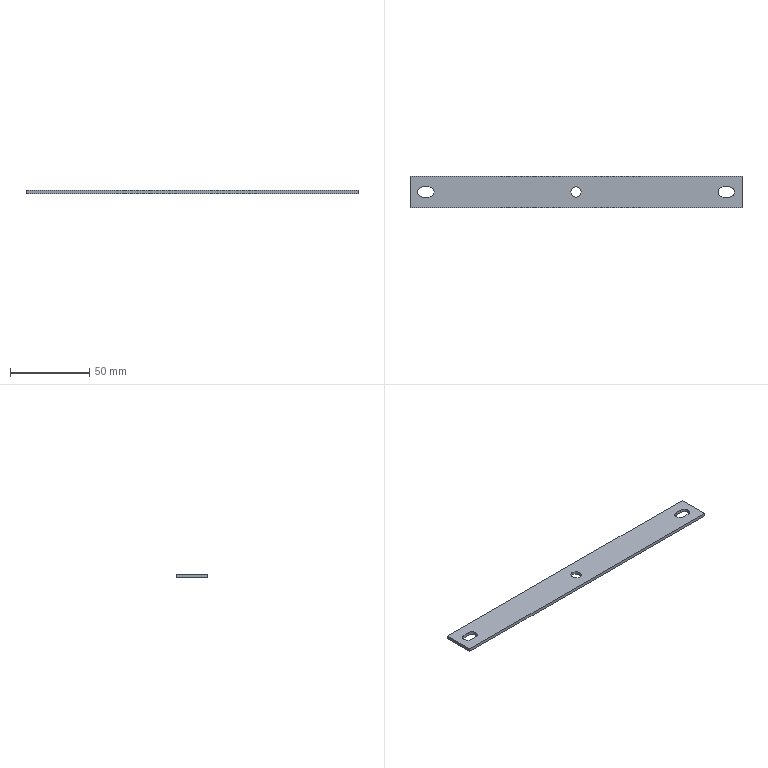Component | SolidWorks | FanFixingPlate-1 | 1 solid | 18 faces | box 210 x 20 x 2 mm | volume 8103 mm3 | plane 10 | cylinder 8 | commonest cylinder face diameters 6.4 x6 6.5 x2
build123d program:
from build123d import *

# Parameters (mm, degrees)
SKETCH1_W           = 210
SKETCH1_H           = 20
BOSS_EXTRUDE1_DEPTH = 1
SKETCH2_R           = 3.25
CUT_EXTRUDE1_DEPTH  = 2


with BuildPart() as part:
    # Sketch1 → Boss-Extrude1 (new, symmetric)
    with BuildSketch(Plane.XY):
        Rectangle(SKETCH1_W, SKETCH1_H)
    extrude(amount=BOSS_EXTRUDE1_DEPTH, both=True)

    # Sketch2 → Cut-Extrude1 (cut)
    with BuildSketch(Plane.XY.offset(1)):
        Circle(SKETCH2_R)
        with BuildLine():
            Line((-97, 3.2), (-93, 3.2))
            ThreePointArc((-93, 3.2), (-89.8, 0), (-93, -3.2))
            Line((-93, -3.2), (-97, -3.2))
            ThreePointArc((-97, -3.2), (-100.2, 0), (-97, 3.2))
        make_face()
        with BuildLine():
            Line((97, 3.2), (93, 3.2))
            ThreePointArc((93, 3.2), (89.8, 0), (93, -3.2))
            Line((93, -3.2), (97, -3.2))
            ThreePointArc((97, -3.2), (100.2, 0), (97, 3.2))
        make_face()
    extrude(amount=-CUT_EXTRUDE1_DEPTH, mode=Mode.SUBTRACT)


solid = part.part

# Placed as in the assembly
solid = solid.moved(Location((254.622, 45.501, 347.013), (0, 0, 0)))
STEP:
#1=COLOUR_RGB('',0.7922,0.8196,0.9333);
#2=FILL_AREA_STYLE_COLOUR('',#1);
#3=FILL_AREA_STYLE('',(#2));
#4=SURFACE_STYLE_FILL_AREA(#3);
#5=SURFACE_SIDE_STYLE('',(#4));
#6=SURFACE_STYLE_USAGE(.BOTH.,#5);
#7=PRESENTATION_STYLE_ASSIGNMENT((#6));
#8=CARTESIAN_POINT('',(13.969,1.791,13.701));
#9=VERTEX_POINT('',#8);
#10=CARTESIAN_POINT('',(13.843,1.665,13.701));
#11=VERTEX_POINT('',#10);
#12=CARTESIAN_POINT('',(13.843,1.791,13.701));
#13=DIRECTION('',(0.,-0.,-1.));
#14=DIRECTION('',(-1.,0.,0.));
#15=AXIS2_PLACEMENT_3D('',#12,#13,#14);
#16=CIRCLE('',#15,0.126);
#17=EDGE_CURVE('',#9,#11,#16,.T.);
#18=ORIENTED_EDGE('',*,*,#17,.F.);
#19=CARTESIAN_POINT('',(13.969,1.791,13.623));
#20=VERTEX_POINT('',#19);
#21=CARTESIAN_POINT('',(13.969,1.791,13.701));
#22=DIRECTION('',(0.,-0.,-1.));
#23=VECTOR('',#22,39.37);
#24=LINE('',#21,#23);
#25=EDGE_CURVE('',#9,#20,#24,.T.);
#26=ORIENTED_EDGE('',*,*,#25,.T.);
#27=CARTESIAN_POINT('',(13.843,1.665,13.623));
#28=VERTEX_POINT('',#27);
#29=CARTESIAN_POINT('',(13.843,1.791,13.623));
#30=DIRECTION('',(0.,-0.,-1.));
#31=DIRECTION('',(-1.,0.,0.));
#32=AXIS2_PLACEMENT_3D('',#29,#30,#31);
#33=CIRCLE('',#32,0.126);
#34=EDGE_CURVE('',#20,#28,#33,.T.);
#35=ORIENTED_EDGE('',*,*,#34,.T.);
#36=CARTESIAN_POINT('',(13.843,1.665,13.701));
#37=DIRECTION('',(0.,-0.,-1.));
#38=VECTOR('',#37,39.37);
#39=LINE('',#36,#38);
#40=EDGE_CURVE('',#11,#28,#39,.T.);
#41=ORIENTED_EDGE('',*,*,#40,.F.);
#42=EDGE_LOOP('',(#18,#26,#35,#41));
#43=FACE_OUTER_BOUND('',#42,.T.);
#44=CARTESIAN_POINT('',(13.843,1.791,13.701));
#45=DIRECTION('',(0.,-0.,-1.));
#46=DIRECTION('',(1.,0.,0.));
#47=AXIS2_PLACEMENT_3D('',#44,#45,#46);
#48=CYLINDRICAL_SURFACE('',#47,0.126);
#49=ADVANCED_FACE('',(#43),#48,.F.);
#50=CARTESIAN_POINT('',(6.489,1.791,13.701));
#51=VERTEX_POINT('',#50);
#52=CARTESIAN_POINT('',(6.363,1.665,13.701));
#53=VERTEX_POINT('',#52);
#54=CARTESIAN_POINT('',(6.363,1.791,13.701));
#55=DIRECTION('',(0.,-0.,-1.));
#56=DIRECTION('',(1.,0.,0.));
#57=AXIS2_PLACEMENT_3D('',#54,#55,#56);
#58=CIRCLE('',#57,0.126);
#59=EDGE_CURVE('',#51,#53,#58,.T.);
#60=ORIENTED_EDGE('',*,*,#59,.F.);
#61=CARTESIAN_POINT('',(6.489,1.791,13.623));
#62=VERTEX_POINT('',#61);
#63=CARTESIAN_POINT('',(6.489,1.791,13.701));
#64=DIRECTION('',(0.,-0.,-1.));
#65=VECTOR('',#64,39.37);
#66=LINE('',#63,#65);
#67=EDGE_CURVE('',#51,#62,#66,.T.);
#68=ORIENTED_EDGE('',*,*,#67,.T.);
#69=CARTESIAN_POINT('',(6.363,1.665,13.623));
#70=VERTEX_POINT('',#69);
#71=CARTESIAN_POINT('',(6.363,1.791,13.623));
#72=DIRECTION('',(0.,-0.,-1.));
#73=DIRECTION('',(1.,0.,0.));
#74=AXIS2_PLACEMENT_3D('',#71,#72,#73);
#75=CIRCLE('',#74,0.126);
#76=EDGE_CURVE('',#62,#70,#75,.T.);
#77=ORIENTED_EDGE('',*,*,#76,.T.);
#78=CARTESIAN_POINT('',(6.363,1.665,13.701));
#79=DIRECTION('',(0.,-0.,-1.));
#80=VECTOR('',#79,39.37);
#81=LINE('',#78,#80);
#82=EDGE_CURVE('',#53,#70,#81,.T.);
#83=ORIENTED_EDGE('',*,*,#82,.F.);
#84=EDGE_LOOP('',(#60,#68,#77,#83));
#85=FACE_OUTER_BOUND('',#84,.T.);
#86=CARTESIAN_POINT('',(6.363,1.791,13.701));
#87=DIRECTION('',(0.,-0.,-1.));
#88=DIRECTION('',(1.,0.,0.));
#89=AXIS2_PLACEMENT_3D('',#86,#87,#88);
#90=CYLINDRICAL_SURFACE('',#89,0.126);
#91=ADVANCED_FACE('',(#85),#90,.F.);
#92=CARTESIAN_POINT('',(9.897,1.791,13.701));
#93=VERTEX_POINT('',#92);
#94=CARTESIAN_POINT('',(10.152,1.791,13.701));
#95=VERTEX_POINT('',#94);
#96=CARTESIAN_POINT('',(10.024,1.791,13.701));
#97=DIRECTION('',(0.,-0.,-1.));
#98=DIRECTION('',(1.,0.,0.));
#99=AXIS2_PLACEMENT_3D('',#96,#97,#98);
#100=CIRCLE('',#99,0.128);
#101=EDGE_CURVE('',#93,#95,#100,.T.);
#102=ORIENTED_EDGE('',*,*,#101,.F.);
#103=CARTESIAN_POINT('',(9.897,1.791,13.623));
#104=VERTEX_POINT('',#103);
#105=CARTESIAN_POINT('',(9.897,1.791,13.701));
#106=DIRECTION('',(0.,-0.,-1.));
#107=VECTOR('',#106,39.37);
#108=LINE('',#105,#107);
#109=EDGE_CURVE('',#93,#104,#108,.T.);
#110=ORIENTED_EDGE('',*,*,#109,.T.);
#111=CARTESIAN_POINT('',(10.152,1.791,13.623));
#112=VERTEX_POINT('',#111);
#113=CARTESIAN_POINT('',(10.024,1.791,13.623));
#114=DIRECTION('',(0.,-0.,-1.));
#115=DIRECTION('',(1.,0.,0.));
#116=AXIS2_PLACEMENT_3D('',#113,#114,#115);
#117=CIRCLE('',#116,0.128);
#118=EDGE_CURVE('',#104,#112,#117,.T.);
#119=ORIENTED_EDGE('',*,*,#118,.T.);
#120=CARTESIAN_POINT('',(10.152,1.791,13.701));
#121=DIRECTION('',(0.,-0.,-1.));
#122=VECTOR('',#121,39.37);
#123=LINE('',#120,#122);
#124=EDGE_CURVE('',#95,#112,#123,.T.);
#125=ORIENTED_EDGE('',*,*,#124,.F.);
#126=EDGE_LOOP('',(#102,#110,#119,#125));
#127=FACE_OUTER_BOUND('',#126,.T.);
#128=CARTESIAN_POINT('',(10.024,1.791,13.701));
#129=DIRECTION('',(0.,-0.,-1.));
#130=DIRECTION('',(1.,0.,0.));
#131=AXIS2_PLACEMENT_3D('',#128,#129,#130);
#132=CYLINDRICAL_SURFACE('',#131,0.128);
#133=ADVANCED_FACE('',(#127),#132,.F.);
#134=CARTESIAN_POINT('',(14.158,2.185,13.701));
#135=VERTEX_POINT('',#134);
#136=CARTESIAN_POINT('',(14.158,1.398,13.701));
#137=VERTEX_POINT('',#136);
#138=CARTESIAN_POINT('',(14.158,1.398,13.701));
#139=DIRECTION('',(-0.,-1.,0.));
#140=VECTOR('',#139,39.37);
#141=LINE('',#138,#140);
#142=EDGE_CURVE('',#135,#137,#141,.T.);
#143=ORIENTED_EDGE('',*,*,#142,.T.);
#144=CARTESIAN_POINT('',(14.158,1.398,13.623));
#145=VERTEX_POINT('',#144);
#146=CARTESIAN_POINT('',(14.158,1.398,13.623));
#147=DIRECTION('',(-0.,0.,1.));
#148=VECTOR('',#147,39.37);
#149=LINE('',#146,#148);
#150=EDGE_CURVE('',#145,#137,#149,.T.);
#151=ORIENTED_EDGE('',*,*,#150,.F.);
#152=CARTESIAN_POINT('',(14.158,2.185,13.623));
#153=VERTEX_POINT('',#152);
#154=CARTESIAN_POINT('',(14.158,1.398,13.623));
#155=DIRECTION('',(-0.,-1.,0.));
#156=VECTOR('',#155,39.37);
#157=LINE('',#154,#156);
#158=EDGE_CURVE('',#153,#145,#157,.T.);
#159=ORIENTED_EDGE('',*,*,#158,.F.);
#160=CARTESIAN_POINT('',(14.158,2.185,13.623));
#161=DIRECTION('',(-0.,0.,1.));
#162=VECTOR('',#161,39.37);
#163=LINE('',#160,#162);
#164=EDGE_CURVE('',#153,#135,#163,.T.);
#165=ORIENTED_EDGE('',*,*,#164,.T.);
#166=EDGE_LOOP('',(#143,#151,#159,#165));
#167=FACE_OUTER_BOUND('',#166,.T.);
#168=CARTESIAN_POINT('',(14.158,1.398,13.623));
#169=DIRECTION('',(-1.,0.,-0.));
#170=DIRECTION('',(0.,-0.,-1.));
#171=AXIS2_PLACEMENT_3D('',#168,#169,#170);
#172=PLANE('',#171);
#173=ADVANCED_FACE('',(#167),#172,.F.);
#174=CARTESIAN_POINT('',(5.891,1.398,13.701));
#175=VERTEX_POINT('',#174);
#176=CARTESIAN_POINT('',(5.891,1.398,13.701));
#177=DIRECTION('',(-1.,0.,-0.));
#178=VECTOR('',#177,39.37);
#179=LINE('',#176,#178);
#180=EDGE_CURVE('',#137,#175,#179,.T.);
#181=ORIENTED_EDGE('',*,*,#180,.T.);
#182=CARTESIAN_POINT('',(5.891,1.398,13.623));
#183=VERTEX_POINT('',#182);
#184=CARTESIAN_POINT('',(5.891,1.398,13.623));
#185=DIRECTION('',(-0.,0.,1.));
#186=VECTOR('',#185,39.37);
#187=LINE('',#184,#186);
#188=EDGE_CURVE('',#183,#175,#187,.T.);
#189=ORIENTED_EDGE('',*,*,#188,.F.);
#190=CARTESIAN_POINT('',(5.891,1.398,13.623));
#191=DIRECTION('',(-1.,0.,-0.));
#192=VECTOR('',#191,39.37);
#193=LINE('',#190,#192);
#194=EDGE_CURVE('',#145,#183,#193,.T.);
#195=ORIENTED_EDGE('',*,*,#194,.F.);
#196=ORIENTED_EDGE('',*,*,#150,.T.);
#197=EDGE_LOOP('',(#181,#189,#195,#196));
#198=FACE_OUTER_BOUND('',#197,.T.);
#199=CARTESIAN_POINT('',(5.891,1.398,13.623));
#200=DIRECTION('',(0.,1.,-0.));
#201=DIRECTION('',(-0.,0.,1.));
#202=AXIS2_PLACEMENT_3D('',#199,#200,#201);
#203=PLANE('',#202);
#204=ADVANCED_FACE('',(#198),#203,.F.);
#205=CARTESIAN_POINT('',(5.891,2.185,13.701));
#206=VERTEX_POINT('',#205);
#207=CARTESIAN_POINT('',(5.891,1.398,13.701));
#208=DIRECTION('',(0.,1.,-0.));
#209=VECTOR('',#208,39.37);
#210=LINE('',#207,#209);
#211=EDGE_CURVE('',#175,#206,#210,.T.);
#212=ORIENTED_EDGE('',*,*,#211,.T.);
#213=CARTESIAN_POINT('',(5.891,2.185,13.623));
#214=VERTEX_POINT('',#213);
#215=CARTESIAN_POINT('',(5.891,2.185,13.623));
#216=DIRECTION('',(-0.,0.,1.));
#217=VECTOR('',#216,39.37);
#218=LINE('',#215,#217);
#219=EDGE_CURVE('',#214,#206,#218,.T.);
#220=ORIENTED_EDGE('',*,*,#219,.F.);
#221=CARTESIAN_POINT('',(5.891,1.398,13.623));
#222=DIRECTION('',(0.,1.,-0.));
#223=VECTOR('',#222,39.37);
#224=LINE('',#221,#223);
#225=EDGE_CURVE('',#183,#214,#224,.T.);
#226=ORIENTED_EDGE('',*,*,#225,.F.);
#227=ORIENTED_EDGE('',*,*,#188,.T.);
#228=EDGE_LOOP('',(#212,#220,#226,#227));
#229=FACE_OUTER_BOUND('',#228,.T.);
#230=CARTESIAN_POINT('',(5.891,1.398,13.623));
#231=DIRECTION('',(1.,-0.,0.));
#232=DIRECTION('',(-0.,0.,1.));
#233=AXIS2_PLACEMENT_3D('',#230,#231,#232);
#234=PLANE('',#233);
#235=ADVANCED_FACE('',(#229),#234,.F.);
#236=CARTESIAN_POINT('',(5.891,2.185,13.701));
#237=DIRECTION('',(1.,-0.,0.));
#238=VECTOR('',#237,39.37);
#239=LINE('',#236,#238);
#240=EDGE_CURVE('',#206,#135,#239,.T.);
#241=ORIENTED_EDGE('',*,*,#240,.T.);
#242=ORIENTED_EDGE('',*,*,#164,.F.);
#243=CARTESIAN_POINT('',(5.891,2.185,13.623));
#244=DIRECTION('',(1.,-0.,0.));
#245=VECTOR('',#244,39.37);
#246=LINE('',#243,#245);
#247=EDGE_CURVE('',#214,#153,#246,.T.);
#248=ORIENTED_EDGE('',*,*,#247,.F.);
#249=ORIENTED_EDGE('',*,*,#219,.T.);
#250=EDGE_LOOP('',(#241,#242,#248,#249));
#251=FACE_OUTER_BOUND('',#250,.T.);
#252=CARTESIAN_POINT('',(5.891,2.185,13.623));
#253=DIRECTION('',(-0.,-1.,0.));
#254=DIRECTION('',(0.,-0.,-1.));
#255=AXIS2_PLACEMENT_3D('',#252,#253,#254);
#256=PLANE('',#255);
#257=ADVANCED_FACE('',(#251),#256,.F.);
#258=CARTESIAN_POINT('',(13.843,1.917,13.623));
#259=VERTEX_POINT('',#258);
#260=CARTESIAN_POINT('',(13.843,1.791,13.623));
#261=DIRECTION('',(0.,-0.,-1.));
#262=DIRECTION('',(-1.,0.,0.));
#263=AXIS2_PLACEMENT_3D('',#260,#261,#262);
#264=CIRCLE('',#263,0.126);
#265=EDGE_CURVE('',#259,#20,#264,.T.);
#266=ORIENTED_EDGE('',*,*,#265,.F.);
#267=CARTESIAN_POINT('',(13.686,1.917,13.623));
#268=VERTEX_POINT('',#267);
#269=CARTESIAN_POINT('',(13.843,1.917,13.623));
#270=DIRECTION('',(1.,0.,0.));
#271=VECTOR('',#270,39.37);
#272=LINE('',#269,#271);
#273=EDGE_CURVE('',#268,#259,#272,.T.);
#274=ORIENTED_EDGE('',*,*,#273,.F.);
#275=CARTESIAN_POINT('',(13.686,1.665,13.623));
#276=VERTEX_POINT('',#275);
#277=CARTESIAN_POINT('',(13.686,1.791,13.623));
#278=DIRECTION('',(0.,-0.,-1.));
#279=DIRECTION('',(-1.,0.,0.));
#280=AXIS2_PLACEMENT_3D('',#277,#278,#279);
#281=CIRCLE('',#280,0.126);
#282=EDGE_CURVE('',#276,#268,#281,.T.);
#283=ORIENTED_EDGE('',*,*,#282,.F.);
#284=CARTESIAN_POINT('',(13.843,1.665,13.623));
#285=DIRECTION('',(-1.,-0.,-0.));
#286=VECTOR('',#285,39.37);
#287=LINE('',#284,#286);
#288=EDGE_CURVE('',#28,#276,#287,.T.);
#289=ORIENTED_EDGE('',*,*,#288,.F.);
#290=ORIENTED_EDGE('',*,*,#34,.F.);
#291=EDGE_LOOP('',(#266,#274,#283,#289,#290));
#292=FACE_BOUND('',#291,.T.);
#293=CARTESIAN_POINT('',(6.206,1.665,13.623));
#294=VERTEX_POINT('',#293);
#295=CARTESIAN_POINT('',(6.206,1.917,13.623));
#296=VERTEX_POINT('',#295);
#297=CARTESIAN_POINT('',(6.206,1.791,13.623));
#298=DIRECTION('',(0.,-0.,-1.));
#299=DIRECTION('',(1.,0.,0.));
#300=AXIS2_PLACEMENT_3D('',#297,#298,#299);
#301=CIRCLE('',#300,0.126);
#302=EDGE_CURVE('',#294,#296,#301,.T.);
#303=ORIENTED_EDGE('',*,*,#302,.F.);
#304=CARTESIAN_POINT('',(6.206,1.665,13.623));
#305=DIRECTION('',(-1.,0.,-0.));
#306=VECTOR('',#305,39.37);
#307=LINE('',#304,#306);
#308=EDGE_CURVE('',#70,#294,#307,.T.);
#309=ORIENTED_EDGE('',*,*,#308,.F.);
#310=ORIENTED_EDGE('',*,*,#76,.F.);
#311=CARTESIAN_POINT('',(6.363,1.917,13.623));
#312=VERTEX_POINT('',#311);
#313=CARTESIAN_POINT('',(6.363,1.791,13.623));
#314=DIRECTION('',(0.,-0.,-1.));
#315=DIRECTION('',(1.,0.,0.));
#316=AXIS2_PLACEMENT_3D('',#313,#314,#315);
#317=CIRCLE('',#316,0.126);
#318=EDGE_CURVE('',#312,#62,#317,.T.);
#319=ORIENTED_EDGE('',*,*,#318,.F.);
#320=CARTESIAN_POINT('',(6.206,1.917,13.623));
#321=DIRECTION('',(1.,-0.,0.));
#322=VECTOR('',#321,39.37);
#323=LINE('',#320,#322);
#324=EDGE_CURVE('',#296,#312,#323,.T.);
#325=ORIENTED_EDGE('',*,*,#324,.F.);
#326=EDGE_LOOP('',(#303,#309,#310,#319,#325));
#327=FACE_BOUND('',#326,.T.);
#328=CARTESIAN_POINT('',(10.024,1.791,13.623));
#329=DIRECTION('',(0.,-0.,-1.));
#330=DIRECTION('',(1.,0.,0.));
#331=AXIS2_PLACEMENT_3D('',#328,#329,#330);
#332=CIRCLE('',#331,0.128);
#333=EDGE_CURVE('',#112,#104,#332,.T.);
#334=ORIENTED_EDGE('',*,*,#333,.F.);
#335=ORIENTED_EDGE('',*,*,#118,.F.);
#336=EDGE_LOOP('',(#334,#335));
#337=FACE_BOUND('',#336,.T.);
#338=ORIENTED_EDGE('',*,*,#158,.T.);
#339=ORIENTED_EDGE('',*,*,#194,.T.);
#340=ORIENTED_EDGE('',*,*,#225,.T.);
#341=ORIENTED_EDGE('',*,*,#247,.T.);
#342=EDGE_LOOP('',(#338,#339,#340,#341));
#343=FACE_OUTER_BOUND('',#342,.T.);
#344=CARTESIAN_POINT('',(14.158,2.185,13.623));
#345=DIRECTION('',(0.,-0.,-1.));
#346=DIRECTION('',(1.,-0.,0.));
#347=AXIS2_PLACEMENT_3D('',#344,#345,#346);
#348=PLANE('',#347);
#349=ADVANCED_FACE('',(#292,#327,#337,#343),#348,.T.);
#350=CARTESIAN_POINT('',(13.686,1.917,13.701));
#351=VERTEX_POINT('',#350);
#352=CARTESIAN_POINT('',(13.843,1.917,13.701));
#353=VERTEX_POINT('',#352);
#354=CARTESIAN_POINT('',(13.843,1.917,13.701));
#355=DIRECTION('',(1.,0.,0.));
#356=VECTOR('',#355,39.37);
#357=LINE('',#354,#356);
#358=EDGE_CURVE('',#351,#353,#357,.T.);
#359=ORIENTED_EDGE('',*,*,#358,.T.);
#360=CARTESIAN_POINT('',(13.843,1.791,13.701));
#361=DIRECTION('',(0.,-0.,-1.));
#362=DIRECTION('',(-1.,0.,0.));
#363=AXIS2_PLACEMENT_3D('',#360,#361,#362);
#364=CIRCLE('',#363,0.126);
#365=EDGE_CURVE('',#353,#9,#364,.T.);
#366=ORIENTED_EDGE('',*,*,#365,.T.);
#367=ORIENTED_EDGE('',*,*,#17,.T.);
#368=CARTESIAN_POINT('',(13.686,1.665,13.701));
#369=VERTEX_POINT('',#368);
#370=CARTESIAN_POINT('',(13.843,1.665,13.701));
#371=DIRECTION('',(-1.,-0.,-0.));
#372=VECTOR('',#371,39.37);
#373=LINE('',#370,#372);
#374=EDGE_CURVE('',#11,#369,#373,.T.);
#375=ORIENTED_EDGE('',*,*,#374,.T.);
#376=CARTESIAN_POINT('',(13.686,1.791,13.701));
#377=DIRECTION('',(0.,-0.,-1.));
#378=DIRECTION('',(-1.,0.,0.));
#379=AXIS2_PLACEMENT_3D('',#376,#377,#378);
#380=CIRCLE('',#379,0.126);
#381=EDGE_CURVE('',#369,#351,#380,.T.);
#382=ORIENTED_EDGE('',*,*,#381,.T.);
#383=EDGE_LOOP('',(#359,#366,#367,#375,#382));
#384=FACE_BOUND('',#383,.T.);
#385=CARTESIAN_POINT('',(6.206,1.665,13.701));
#386=VERTEX_POINT('',#385);
#387=CARTESIAN_POINT('',(6.206,1.665,13.701));
#388=DIRECTION('',(-1.,0.,-0.));
#389=VECTOR('',#388,39.37);
#390=LINE('',#387,#389);
#391=EDGE_CURVE('',#53,#386,#390,.T.);
#392=ORIENTED_EDGE('',*,*,#391,.T.);
#393=CARTESIAN_POINT('',(6.206,1.917,13.701));
#394=VERTEX_POINT('',#393);
#395=CARTESIAN_POINT('',(6.206,1.791,13.701));
#396=DIRECTION('',(0.,-0.,-1.));
#397=DIRECTION('',(1.,0.,0.));
#398=AXIS2_PLACEMENT_3D('',#395,#396,#397);
#399=CIRCLE('',#398,0.126);
#400=EDGE_CURVE('',#386,#394,#399,.T.);
#401=ORIENTED_EDGE('',*,*,#400,.T.);
#402=CARTESIAN_POINT('',(6.363,1.917,13.701));
#403=VERTEX_POINT('',#402);
#404=CARTESIAN_POINT('',(6.206,1.917,13.701));
#405=DIRECTION('',(1.,-0.,0.));
#406=VECTOR('',#405,39.37);
#407=LINE('',#404,#406);
#408=EDGE_CURVE('',#394,#403,#407,.T.);
#409=ORIENTED_EDGE('',*,*,#408,.T.);
#410=CARTESIAN_POINT('',(6.363,1.791,13.701));
#411=DIRECTION('',(0.,-0.,-1.));
#412=DIRECTION('',(1.,0.,0.));
#413=AXIS2_PLACEMENT_3D('',#410,#411,#412);
#414=CIRCLE('',#413,0.126);
#415=EDGE_CURVE('',#403,#51,#414,.T.);
#416=ORIENTED_EDGE('',*,*,#415,.T.);
#417=ORIENTED_EDGE('',*,*,#59,.T.);
#418=EDGE_LOOP('',(#392,#401,#409,#416,#417));
#419=FACE_BOUND('',#418,.T.);
#420=CARTESIAN_POINT('',(10.024,1.791,13.701));
#421=DIRECTION('',(0.,-0.,-1.));
#422=DIRECTION('',(1.,0.,0.));
#423=AXIS2_PLACEMENT_3D('',#420,#421,#422);
#424=CIRCLE('',#423,0.128);
#425=EDGE_CURVE('',#95,#93,#424,.T.);
#426=ORIENTED_EDGE('',*,*,#425,.T.);
#427=ORIENTED_EDGE('',*,*,#101,.T.);
#428=EDGE_LOOP('',(#426,#427));
#429=FACE_BOUND('',#428,.T.);
#430=ORIENTED_EDGE('',*,*,#142,.F.);
#431=ORIENTED_EDGE('',*,*,#240,.F.);
#432=ORIENTED_EDGE('',*,*,#211,.F.);
#433=ORIENTED_EDGE('',*,*,#180,.F.);
#434=EDGE_LOOP('',(#430,#431,#432,#433));
#435=FACE_OUTER_BOUND('',#434,.T.);
#436=CARTESIAN_POINT('',(14.158,2.185,13.701));
#437=DIRECTION('',(0.,-0.,-1.));
#438=DIRECTION('',(1.,-0.,0.));
#439=AXIS2_PLACEMENT_3D('',#436,#437,#438);
#440=PLANE('',#439);
#441=ADVANCED_FACE('',(#384,#419,#429,#435),#440,.F.);
#442=ORIENTED_EDGE('',*,*,#109,.F.);
#443=ORIENTED_EDGE('',*,*,#425,.F.);
#444=ORIENTED_EDGE('',*,*,#124,.T.);
#445=ORIENTED_EDGE('',*,*,#333,.T.);
#446=EDGE_LOOP('',(#442,#443,#444,#445));
#447=FACE_OUTER_BOUND('',#446,.T.);
#448=CARTESIAN_POINT('',(10.024,1.791,13.701));
#449=DIRECTION('',(0.,-0.,-1.));
#450=DIRECTION('',(1.,0.,0.));
#451=AXIS2_PLACEMENT_3D('',#448,#449,#450);
#452=CYLINDRICAL_SURFACE('',#451,0.128);
#453=ADVANCED_FACE('',(#447),#452,.F.);
#454=ORIENTED_EDGE('',*,*,#302,.T.);
#455=CARTESIAN_POINT('',(6.206,1.917,13.701));
#456=DIRECTION('',(0.,-0.,-1.));
#457=VECTOR('',#456,39.37);
#458=LINE('',#455,#457);
#459=EDGE_CURVE('',#394,#296,#458,.T.);
#460=ORIENTED_EDGE('',*,*,#459,.F.);
#461=ORIENTED_EDGE('',*,*,#400,.F.);
#462=CARTESIAN_POINT('',(6.206,1.665,13.701));
#463=DIRECTION('',(0.,-0.,-1.));
#464=VECTOR('',#463,39.37);
#465=LINE('',#462,#464);
#466=EDGE_CURVE('',#386,#294,#465,.T.);
#467=ORIENTED_EDGE('',*,*,#466,.T.);
#468=EDGE_LOOP('',(#454,#460,#461,#467));
#469=FACE_OUTER_BOUND('',#468,.T.);
#470=CARTESIAN_POINT('',(6.206,1.791,13.701));
#471=DIRECTION('',(0.,-0.,-1.));
#472=DIRECTION('',(1.,0.,0.));
#473=AXIS2_PLACEMENT_3D('',#470,#471,#472);
#474=CYLINDRICAL_SURFACE('',#473,0.126);
#475=ADVANCED_FACE('',(#469),#474,.F.);
#476=ORIENTED_EDGE('',*,*,#308,.T.);
#477=ORIENTED_EDGE('',*,*,#466,.F.);
#478=ORIENTED_EDGE('',*,*,#391,.F.);
#479=ORIENTED_EDGE('',*,*,#82,.T.);
#480=EDGE_LOOP('',(#476,#477,#478,#479));
#481=FACE_OUTER_BOUND('',#480,.T.);
#482=CARTESIAN_POINT('',(6.206,1.665,13.701));
#483=DIRECTION('',(-0.,-1.,0.));
#484=DIRECTION('',(-1.,0.,-0.));
#485=AXIS2_PLACEMENT_3D('',#482,#483,#484);
#486=PLANE('',#485);
#487=ADVANCED_FACE('',(#481),#486,.F.);
#488=ORIENTED_EDGE('',*,*,#67,.F.);
#489=ORIENTED_EDGE('',*,*,#415,.F.);
#490=CARTESIAN_POINT('',(6.363,1.917,13.701));
#491=DIRECTION('',(0.,-0.,-1.));
#492=VECTOR('',#491,39.37);
#493=LINE('',#490,#492);
#494=EDGE_CURVE('',#403,#312,#493,.T.);
#495=ORIENTED_EDGE('',*,*,#494,.T.);
#496=ORIENTED_EDGE('',*,*,#318,.T.);
#497=EDGE_LOOP('',(#488,#489,#495,#496));
#498=FACE_OUTER_BOUND('',#497,.T.);
#499=CARTESIAN_POINT('',(6.363,1.791,13.701));
#500=DIRECTION('',(0.,-0.,-1.));
#501=DIRECTION('',(1.,0.,0.));
#502=AXIS2_PLACEMENT_3D('',#499,#500,#501);
#503=CYLINDRICAL_SURFACE('',#502,0.126);
#504=ADVANCED_FACE('',(#498),#503,.F.);
#505=ORIENTED_EDGE('',*,*,#324,.T.);
#506=ORIENTED_EDGE('',*,*,#494,.F.);
#507=ORIENTED_EDGE('',*,*,#408,.F.);
#508=ORIENTED_EDGE('',*,*,#459,.T.);
#509=EDGE_LOOP('',(#505,#506,#507,#508));
#510=FACE_OUTER_BOUND('',#509,.T.);
#511=CARTESIAN_POINT('',(6.206,1.917,13.701));
#512=DIRECTION('',(0.,1.,-0.));
#513=DIRECTION('',(1.,-0.,0.));
#514=AXIS2_PLACEMENT_3D('',#511,#512,#513);
#515=PLANE('',#514);
#516=ADVANCED_FACE('',(#510),#515,.F.);
#517=ORIENTED_EDGE('',*,*,#25,.F.);
#518=ORIENTED_EDGE('',*,*,#365,.F.);
#519=CARTESIAN_POINT('',(13.843,1.917,13.701));
#520=DIRECTION('',(0.,-0.,-1.));
#521=VECTOR('',#520,39.37);
#522=LINE('',#519,#521);
#523=EDGE_CURVE('',#353,#259,#522,.T.);
#524=ORIENTED_EDGE('',*,*,#523,.T.);
#525=ORIENTED_EDGE('',*,*,#265,.T.);
#526=EDGE_LOOP('',(#517,#518,#524,#525));
#527=FACE_OUTER_BOUND('',#526,.T.);
#528=CARTESIAN_POINT('',(13.843,1.791,13.701));
#529=DIRECTION('',(0.,-0.,-1.));
#530=DIRECTION('',(1.,0.,0.));
#531=AXIS2_PLACEMENT_3D('',#528,#529,#530);
#532=CYLINDRICAL_SURFACE('',#531,0.126);
#533=ADVANCED_FACE('',(#527),#532,.F.);
#534=ORIENTED_EDGE('',*,*,#273,.T.);
#535=ORIENTED_EDGE('',*,*,#523,.F.);
#536=ORIENTED_EDGE('',*,*,#358,.F.);
#537=CARTESIAN_POINT('',(13.686,1.917,13.701));
#538=DIRECTION('',(0.,-0.,-1.));
#539=VECTOR('',#538,39.37);
#540=LINE('',#537,#539);
#541=EDGE_CURVE('',#351,#268,#540,.T.);
#542=ORIENTED_EDGE('',*,*,#541,.T.);
#543=EDGE_LOOP('',(#534,#535,#536,#542));
#544=FACE_OUTER_BOUND('',#543,.T.);
#545=CARTESIAN_POINT('',(13.843,1.917,13.701));
#546=DIRECTION('',(-0.,1.,-0.));
#547=DIRECTION('',(1.,0.,0.));
#548=AXIS2_PLACEMENT_3D('',#545,#546,#547);
#549=PLANE('',#548);
#550=ADVANCED_FACE('',(#544),#549,.F.);
#551=ORIENTED_EDGE('',*,*,#282,.T.);
#552=ORIENTED_EDGE('',*,*,#541,.F.);
#553=ORIENTED_EDGE('',*,*,#381,.F.);
#554=CARTESIAN_POINT('',(13.686,1.665,13.701));
#555=DIRECTION('',(0.,-0.,-1.));
#556=VECTOR('',#555,39.37);
#557=LINE('',#554,#556);
#558=EDGE_CURVE('',#369,#276,#557,.T.);
#559=ORIENTED_EDGE('',*,*,#558,.T.);
#560=EDGE_LOOP('',(#551,#552,#553,#559));
#561=FACE_OUTER_BOUND('',#560,.T.);
#562=CARTESIAN_POINT('',(13.686,1.791,13.701));
#563=DIRECTION('',(0.,-0.,-1.));
#564=DIRECTION('',(1.,0.,0.));
#565=AXIS2_PLACEMENT_3D('',#562,#563,#564);
#566=CYLINDRICAL_SURFACE('',#565,0.126);
#567=ADVANCED_FACE('',(#561),#566,.F.);
#568=ORIENTED_EDGE('',*,*,#288,.T.);
#569=ORIENTED_EDGE('',*,*,#558,.F.);
#570=ORIENTED_EDGE('',*,*,#374,.F.);
#571=ORIENTED_EDGE('',*,*,#40,.T.);
#572=EDGE_LOOP('',(#568,#569,#570,#571));
#573=FACE_OUTER_BOUND('',#572,.T.);
#574=CARTESIAN_POINT('',(13.843,1.665,13.701));
#575=DIRECTION('',(0.,-1.,0.));
#576=DIRECTION('',(-1.,-0.,-0.));
#577=AXIS2_PLACEMENT_3D('',#574,#575,#576);
#578=PLANE('',#577);
#579=ADVANCED_FACE('',(#573),#578,.F.);
#580=CLOSED_SHELL('',(#49,#91,#133,#173,#204,#235,#257,#349,#441,#453,#475,#487,#504,#516,#533,#550,#567,#579));
#581=MANIFOLD_SOLID_BREP('',#580);
#582=STYLED_ITEM('',(#7),#581);
#583=(LENGTH_UNIT()NAMED_UNIT(*)SI_UNIT($,.METRE.));
#584=LENGTH_MEASURE_WITH_UNIT(LENGTH_MEASURE(0.0254),#583);
#585=DIMENSIONAL_EXPONENTS(1.,0.,0.,0.,0.,0.,0.);
#586=(CONVERSION_BASED_UNIT('',#584)LENGTH_UNIT()NAMED_UNIT(#585));
#587=UNCERTAINTY_MEASURE_WITH_UNIT(LENGTH_MEASURE(0.00001),#586,'','');
#588=(NAMED_UNIT(*)PLANE_ANGLE_UNIT()SI_UNIT($,.RADIAN.));
#589=(NAMED_UNIT(*)SI_UNIT($,.STERADIAN.)SOLID_ANGLE_UNIT());
#590=(GEOMETRIC_REPRESENTATION_CONTEXT(3)GLOBAL_UNCERTAINTY_ASSIGNED_CONTEXT((#587))GLOBAL_UNIT_ASSIGNED_CONTEXT((#586,#588,#589))REPRESENTATION_CONTEXT('',''));
#591=MECHANICAL_DESIGN_GEOMETRIC_PRESENTATION_REPRESENTATION('',(#582),#590);
#592=PRESENTATION_LAYER_ASSIGNMENT('','',(#582));
#593=CARTESIAN_POINT('',(0.,0.,0.));
#594=DIRECTION('',(0.,0.,1.));
#595=DIRECTION('',(1.,0.,0.));
#596=AXIS2_PLACEMENT_3D('',#593,#594,#595);
#597=(LENGTH_UNIT()NAMED_UNIT(*)SI_UNIT($,.METRE.));
#598=LENGTH_MEASURE_WITH_UNIT(LENGTH_MEASURE(0.0254),#597);
#599=DIMENSIONAL_EXPONENTS(1.,0.,0.,0.,0.,0.,0.);
#600=(CONVERSION_BASED_UNIT('',#598)LENGTH_UNIT()NAMED_UNIT(#599));
#601=UNCERTAINTY_MEASURE_WITH_UNIT(LENGTH_MEASURE(0.00001),#600,'','');
#602=(NAMED_UNIT(*)PLANE_ANGLE_UNIT()SI_UNIT($,.RADIAN.));
#603=(NAMED_UNIT(*)SI_UNIT($,.STERADIAN.)SOLID_ANGLE_UNIT());
#604=(GEOMETRIC_REPRESENTATION_CONTEXT(3)GLOBAL_UNCERTAINTY_ASSIGNED_CONTEXT((#601))GLOBAL_UNIT_ASSIGNED_CONTEXT((#600,#602,#603))REPRESENTATION_CONTEXT('',''));
#605=ADVANCED_BREP_SHAPE_REPRESENTATION('',(#581,#596),#604);